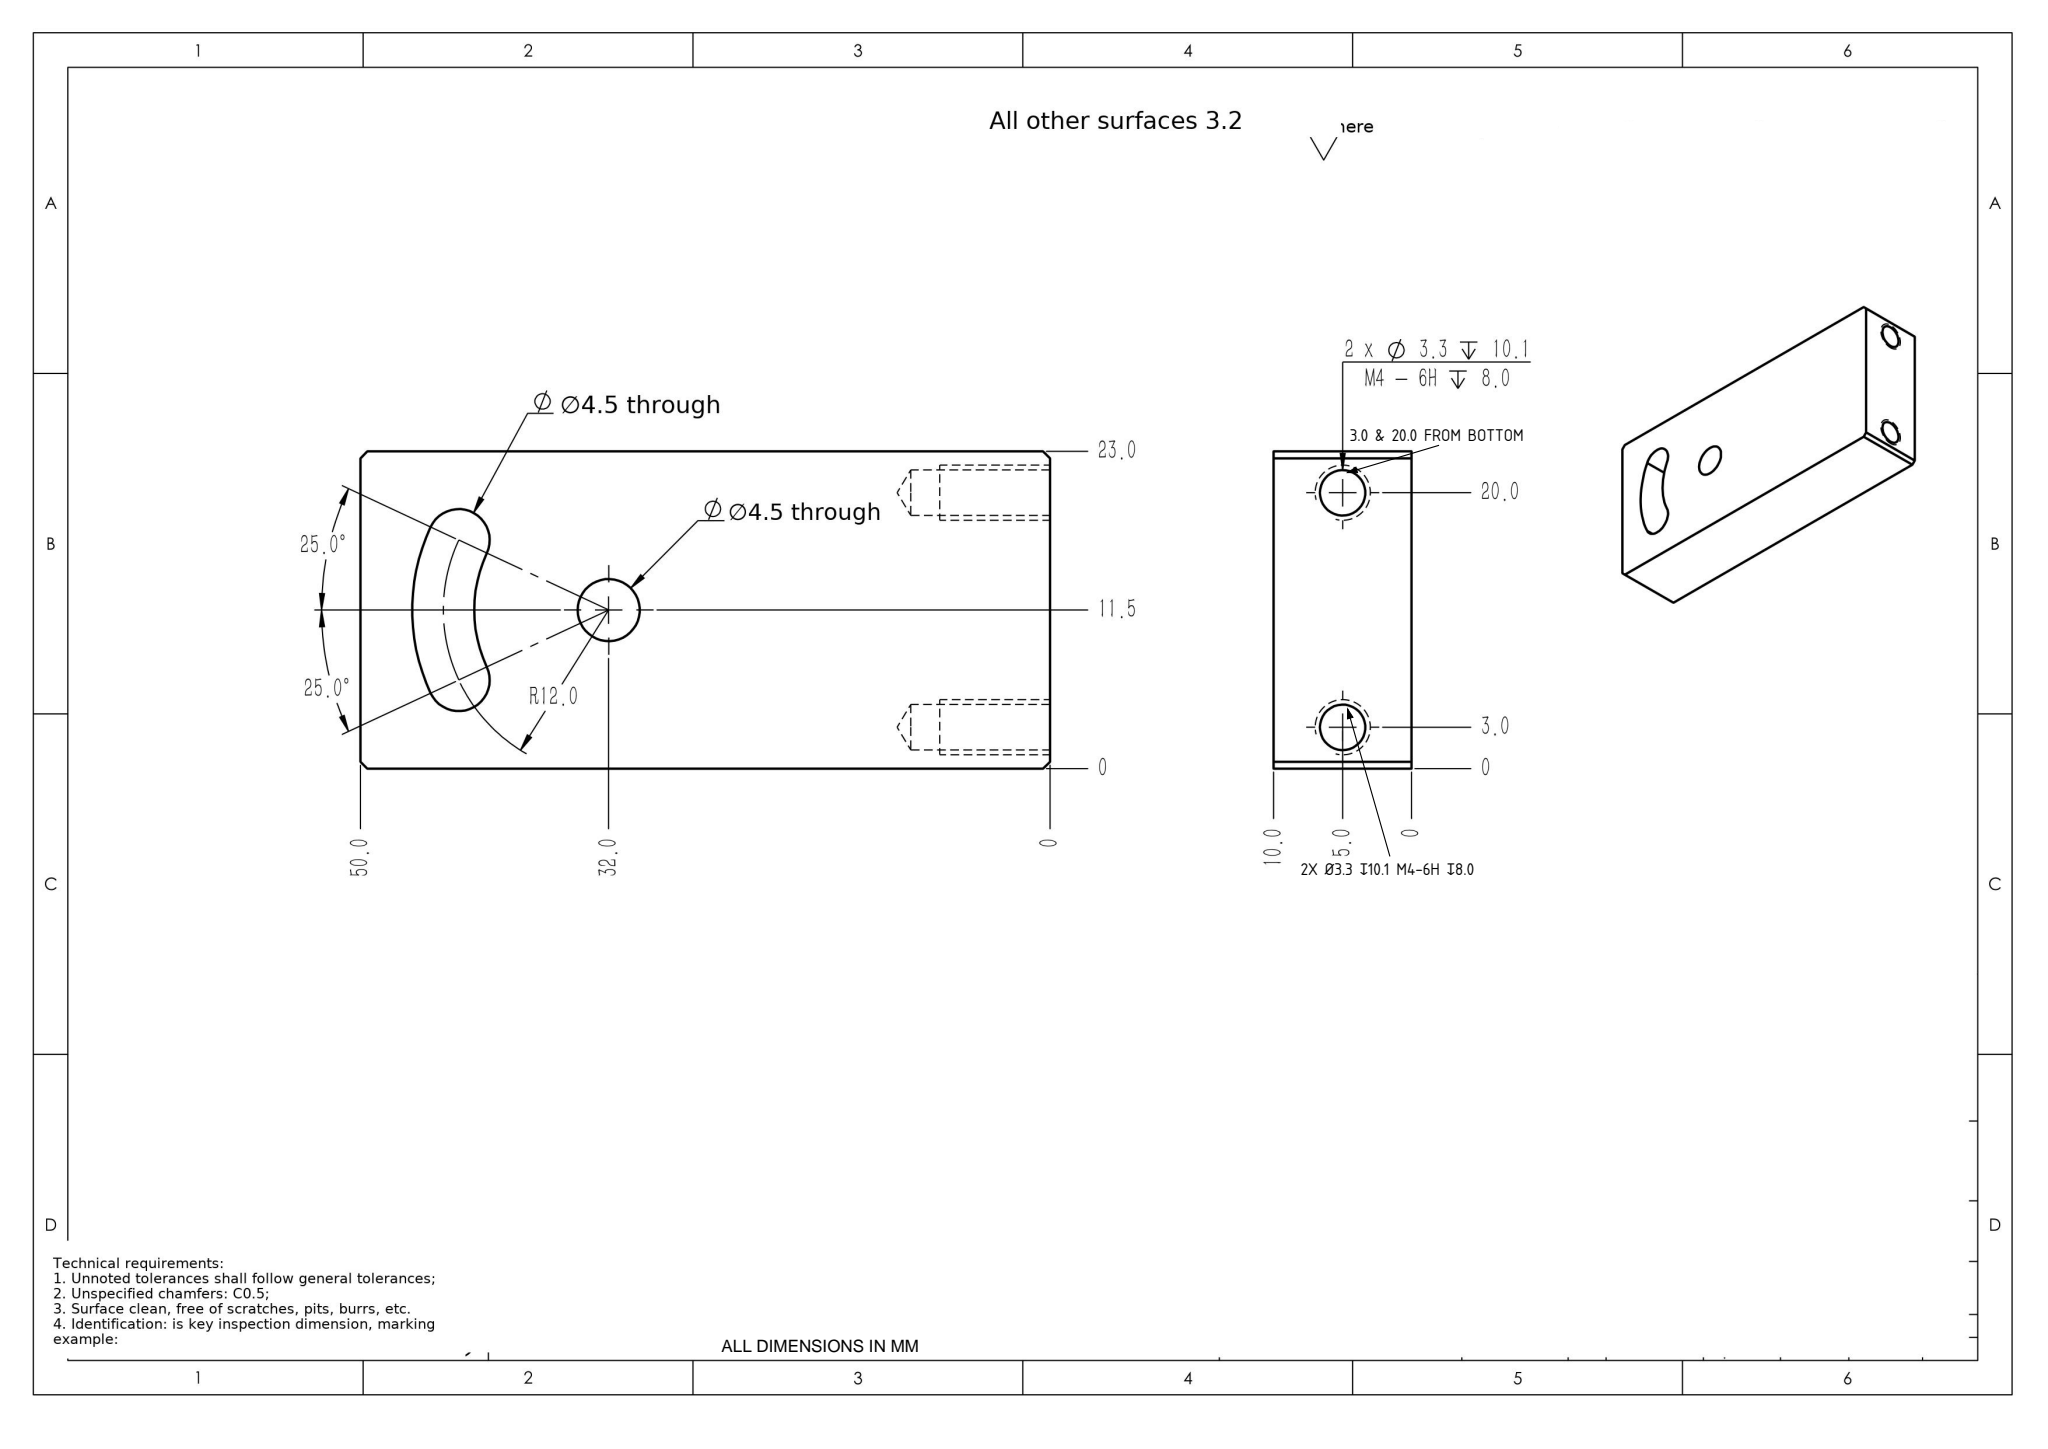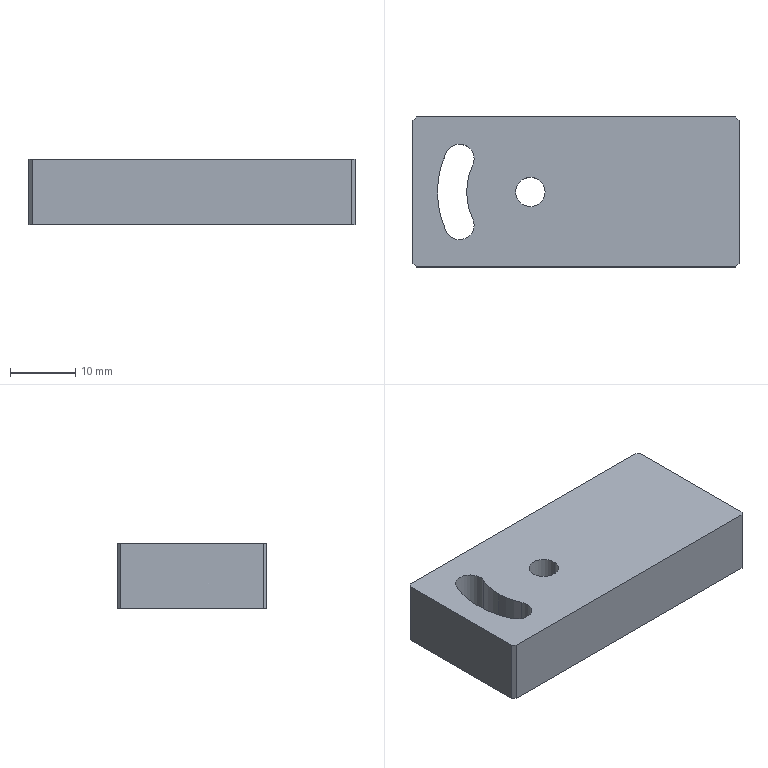Part | SolidWorks | mm | material POM | 1 solid | 26 faces | box 50 x 23 x 10 mm | volume 10527 mm3 | cylinder 12 | plane 10 | cone 4 | commonest cylinder face diameters 4.5 x4 3.3 x4 19.5 x2 28.5 x2
Drawing notes:
2X Ø3.3 DP 10.1, M4-6H DP 8.0 IN END FACE (NOT 4X) | from the solid: Only two Ø3.3 x-axis bores exist: at Y20.0/Z5.0 and Y3.0/Z5.0, from X39.9 to X50.0 (depth 10.1); 118° drill points at X38.9
TAPPED HOLES AT 3.0 & 20.0 FROM BOTTOM, 5.0 FROM FACE | from the solid: hole/bore 3.3 axis x at [y=20.0,z=5.0] and [y=3.0,z=5.0]; bbox 50x23x10
build123d program:
from build123d import *

# Parameters (mm, degrees)
SKETCH1_W             = 50
SKETCH1_H             = 23
BOSS_EXTRUDE1_DEPTH   = 10
M4_TAPPED_HOLE1_D     = 3.3
M4_TAPPED_HOLE1_DEPTH = 10.1
M4_TAPPED_HOLE1_TIP   = 0.9914
SKETCH4_R             = 2.25
CUT_EXTRUDE1_DEPTH    = 30.279
CUT_EXTRUDE2_DEPTH    = 30.279
CHAMFER1_SIZE         = 0.5


with BuildPart() as part:
    # Sketch1 → Boss-Extrude1 (new body)
    with BuildSketch(Plane.XY):
        Rectangle(SKETCH1_W, SKETCH1_H)
    extrude(amount=BOSS_EXTRUDE1_DEPTH)

    # M4 Tapped Hole1
    with Locations(Plane(origin=(25, 0, 0), x_dir=(0, 0, -1), z_dir=(1, 0, 0))):
        with Locations((-5, -8.5), (-5, 8.5)):
            Hole(M4_TAPPED_HOLE1_D / 2, depth=M4_TAPPED_HOLE1_DEPTH)
            with Locations((0, 0, -(M4_TAPPED_HOLE1_DEPTH + M4_TAPPED_HOLE1_TIP / 2))):  # 118° drill point
                Cone(0, M4_TAPPED_HOLE1_D / 2, M4_TAPPED_HOLE1_TIP, mode=Mode.SUBTRACT)

    # Sketch4 → Cut-Extrude1 (cut, through all)
    with BuildSketch(Plane(origin=(0, 0, 0), x_dir=(-1, 0, 0), z_dir=(0, 0, -1))):
        with Locations((7, 0)):
            Circle(SKETCH4_R)
    extrude(amount=-CUT_EXTRUDE1_DEPTH, mode=Mode.SUBTRACT)

    # Sketch5 → Cut-Extrude2 (cut, through all)
    with BuildSketch(Plane(origin=(0, 0, 0), x_dir=(-1, 0, 0), z_dir=(0, 0, -1))):
        with BuildLine():
            ThreePointArc((15.837, -4.121), (16.925, -7.111), (19.915, -6.022))
            ThreePointArc((19.915, -6.022), (21.25, 0), (19.915, 6.022))
            ThreePointArc((19.915, 6.022), (16.925, 7.111), (15.837, 4.121))
            ThreePointArc((15.837, 4.121), (16.75, 0), (15.837, -4.121))
        make_face()
    extrude(amount=-CUT_EXTRUDE2_DEPTH, mode=Mode.SUBTRACT)

    # Chamfer1
    chamfer1_edges = [part.edges().sort_by_distance(p)[0] for p in [
        (25, -11.5, 5),
        (25, 11.5, 5),
        (-25, 11.5, 5),
        (-25, -11.5, 5),
    ]]
    chamfer(chamfer1_edges, length=CHAMFER1_SIZE)


solid = part.part
STEP:
#1=CARTESIAN_POINT('',(-16.75,0.,10.));
#2=VERTEX_POINT('',#1);
#3=CARTESIAN_POINT('',(-15.837,-4.121,10.));
#4=VERTEX_POINT('',#3);
#5=CARTESIAN_POINT('',(-7.,0.,10.));
#6=DIRECTION('',(0.,0.,1.));
#7=DIRECTION('',(-1.,0.,0.));
#8=AXIS2_PLACEMENT_3D('',#5,#6,#7);
#9=CIRCLE('',#8,9.75);
#10=EDGE_CURVE('',#2,#4,#9,.T.);
#11=ORIENTED_EDGE('',*,*,#10,.F.);
#12=CARTESIAN_POINT('',(-16.75,0.,0.));
#13=VERTEX_POINT('',#12);
#14=CARTESIAN_POINT('',(-16.75,0.,10.));
#15=DIRECTION('',(0.,0.,-1.));
#16=VECTOR('',#15,1000.);
#17=LINE('',#14,#16);
#18=EDGE_CURVE('',#2,#13,#17,.T.);
#19=ORIENTED_EDGE('',*,*,#18,.T.);
#20=CARTESIAN_POINT('',(-15.837,-4.121,0.));
#21=VERTEX_POINT('',#20);
#22=CARTESIAN_POINT('',(-7.,0.,0.));
#23=DIRECTION('',(0.,0.,1.));
#24=DIRECTION('',(-1.,0.,0.));
#25=AXIS2_PLACEMENT_3D('',#22,#23,#24);
#26=CIRCLE('',#25,9.75);
#27=EDGE_CURVE('',#13,#21,#26,.T.);
#28=ORIENTED_EDGE('',*,*,#27,.T.);
#29=CARTESIAN_POINT('',(-15.837,-4.121,10.));
#30=DIRECTION('',(0.,0.,-1.));
#31=VECTOR('',#30,1000.);
#32=LINE('',#29,#31);
#33=EDGE_CURVE('',#4,#21,#32,.T.);
#34=ORIENTED_EDGE('',*,*,#33,.F.);
#35=EDGE_LOOP('',(#11,#19,#28,#34));
#36=FACE_OUTER_BOUND('',#35,.T.);
#37=CARTESIAN_POINT('',(-7.,0.,10.));
#38=DIRECTION('',(0.,0.,-1.));
#39=DIRECTION('',(-1.,0.,0.));
#40=AXIS2_PLACEMENT_3D('',#37,#38,#39);
#41=CYLINDRICAL_SURFACE('',#40,9.75);
#42=ADVANCED_FACE('',(#36),#41,.T.);
#43=CARTESIAN_POINT('',(-21.25,0.,10.));
#44=VERTEX_POINT('',#43);
#45=CARTESIAN_POINT('',(-19.915,6.022,10.));
#46=VERTEX_POINT('',#45);
#47=CARTESIAN_POINT('',(-7.,0.,10.));
#48=DIRECTION('',(0.,0.,-1.));
#49=DIRECTION('',(-1.,0.,0.));
#50=AXIS2_PLACEMENT_3D('',#47,#48,#49);
#51=CIRCLE('',#50,14.25);
#52=EDGE_CURVE('',#44,#46,#51,.T.);
#53=ORIENTED_EDGE('',*,*,#52,.F.);
#54=CARTESIAN_POINT('',(-21.25,0.,0.));
#55=VERTEX_POINT('',#54);
#56=CARTESIAN_POINT('',(-21.25,0.,10.));
#57=DIRECTION('',(0.,0.,-1.));
#58=VECTOR('',#57,1000.);
#59=LINE('',#56,#58);
#60=EDGE_CURVE('',#44,#55,#59,.T.);
#61=ORIENTED_EDGE('',*,*,#60,.T.);
#62=CARTESIAN_POINT('',(-19.915,6.022,0.));
#63=VERTEX_POINT('',#62);
#64=CARTESIAN_POINT('',(-7.,0.,0.));
#65=DIRECTION('',(0.,0.,-1.));
#66=DIRECTION('',(-1.,0.,0.));
#67=AXIS2_PLACEMENT_3D('',#64,#65,#66);
#68=CIRCLE('',#67,14.25);
#69=EDGE_CURVE('',#55,#63,#68,.T.);
#70=ORIENTED_EDGE('',*,*,#69,.T.);
#71=CARTESIAN_POINT('',(-19.915,6.022,10.));
#72=DIRECTION('',(0.,0.,-1.));
#73=VECTOR('',#72,1000.);
#74=LINE('',#71,#73);
#75=EDGE_CURVE('',#46,#63,#74,.T.);
#76=ORIENTED_EDGE('',*,*,#75,.F.);
#77=EDGE_LOOP('',(#53,#61,#70,#76));
#78=FACE_OUTER_BOUND('',#77,.T.);
#79=CARTESIAN_POINT('',(-7.,0.,10.));
#80=DIRECTION('',(0.,0.,-1.));
#81=DIRECTION('',(-1.,0.,0.));
#82=AXIS2_PLACEMENT_3D('',#79,#80,#81);
#83=CYLINDRICAL_SURFACE('',#82,14.25);
#84=ADVANCED_FACE('',(#78),#83,.F.);
#85=CARTESIAN_POINT('',(-4.75,0.,10.));
#86=VERTEX_POINT('',#85);
#87=CARTESIAN_POINT('',(-9.25,0.,10.));
#88=VERTEX_POINT('',#87);
#89=CARTESIAN_POINT('',(-7.,0.,10.));
#90=DIRECTION('',(0.,0.,-1.));
#91=DIRECTION('',(-1.,0.,0.));
#92=AXIS2_PLACEMENT_3D('',#89,#90,#91);
#93=CIRCLE('',#92,2.25);
#94=EDGE_CURVE('',#86,#88,#93,.T.);
#95=ORIENTED_EDGE('',*,*,#94,.F.);
#96=CARTESIAN_POINT('',(-4.75,0.,0.));
#97=VERTEX_POINT('',#96);
#98=CARTESIAN_POINT('',(-4.75,0.,10.));
#99=DIRECTION('',(0.,0.,-1.));
#100=VECTOR('',#99,1000.);
#101=LINE('',#98,#100);
#102=EDGE_CURVE('',#86,#97,#101,.T.);
#103=ORIENTED_EDGE('',*,*,#102,.T.);
#104=CARTESIAN_POINT('',(-9.25,0.,0.));
#105=VERTEX_POINT('',#104);
#106=CARTESIAN_POINT('',(-7.,0.,0.));
#107=DIRECTION('',(0.,0.,-1.));
#108=DIRECTION('',(-1.,0.,0.));
#109=AXIS2_PLACEMENT_3D('',#106,#107,#108);
#110=CIRCLE('',#109,2.25);
#111=EDGE_CURVE('',#97,#105,#110,.T.);
#112=ORIENTED_EDGE('',*,*,#111,.T.);
#113=CARTESIAN_POINT('',(-9.25,0.,10.));
#114=DIRECTION('',(0.,0.,-1.));
#115=VECTOR('',#114,1000.);
#116=LINE('',#113,#115);
#117=EDGE_CURVE('',#88,#105,#116,.T.);
#118=ORIENTED_EDGE('',*,*,#117,.F.);
#119=EDGE_LOOP('',(#95,#103,#112,#118));
#120=FACE_OUTER_BOUND('',#119,.T.);
#121=CARTESIAN_POINT('',(-7.,0.,10.));
#122=DIRECTION('',(0.,0.,-1.));
#123=DIRECTION('',(-1.,0.,0.));
#124=AXIS2_PLACEMENT_3D('',#121,#122,#123);
#125=CYLINDRICAL_SURFACE('',#124,2.25);
#126=ADVANCED_FACE('',(#120),#125,.F.);
#127=CARTESIAN_POINT('',(14.9,-8.5,6.65));
#128=VERTEX_POINT('',#127);
#129=CARTESIAN_POINT('',(14.9,-8.5,3.35));
#130=VERTEX_POINT('',#129);
#131=CARTESIAN_POINT('',(14.9,-8.5,5.));
#132=DIRECTION('',(1.,0.,0.));
#133=DIRECTION('',(0.,0.,-1.));
#134=AXIS2_PLACEMENT_3D('',#131,#132,#133);
#135=CIRCLE('',#134,1.65);
#136=EDGE_CURVE('',#128,#130,#135,.T.);
#137=ORIENTED_EDGE('',*,*,#136,.F.);
#138=CARTESIAN_POINT('',(25.,-8.5,6.65));
#139=VERTEX_POINT('',#138);
#140=CARTESIAN_POINT('',(25.,-8.5,6.65));
#141=DIRECTION('',(1.,0.,0.));
#142=VECTOR('',#141,1000.);
#143=LINE('',#140,#142);
#144=EDGE_CURVE('',#128,#139,#143,.T.);
#145=ORIENTED_EDGE('',*,*,#144,.T.);
#146=CARTESIAN_POINT('',(25.,-8.5,3.35));
#147=VERTEX_POINT('',#146);
#148=CARTESIAN_POINT('',(25.,-8.5,5.));
#149=DIRECTION('',(1.,0.,0.));
#150=DIRECTION('',(0.,0.,-1.));
#151=AXIS2_PLACEMENT_3D('',#148,#149,#150);
#152=CIRCLE('',#151,1.65);
#153=EDGE_CURVE('',#139,#147,#152,.T.);
#154=ORIENTED_EDGE('',*,*,#153,.T.);
#155=CARTESIAN_POINT('',(25.,-8.5,3.35));
#156=DIRECTION('',(1.,0.,0.));
#157=VECTOR('',#156,1000.);
#158=LINE('',#155,#157);
#159=EDGE_CURVE('',#130,#147,#158,.T.);
#160=ORIENTED_EDGE('',*,*,#159,.F.);
#161=EDGE_LOOP('',(#137,#145,#154,#160));
#162=FACE_OUTER_BOUND('',#161,.T.);
#163=CARTESIAN_POINT('',(25.,-8.5,5.));
#164=DIRECTION('',(1.,0.,0.));
#165=DIRECTION('',(0.,0.,-1.));
#166=AXIS2_PLACEMENT_3D('',#163,#164,#165);
#167=CYLINDRICAL_SURFACE('',#166,1.65);
#168=ADVANCED_FACE('',(#162),#167,.F.);
#169=CARTESIAN_POINT('',(13.909,-8.5,5.));
#170=VERTEX_POINT('',#169);
#171=CARTESIAN_POINT('',(14.9,-8.5,3.35));
#172=DIRECTION('',(0.515,0.,-0.8572));
#173=VECTOR('',#172,1000.);
#174=LINE('',#171,#173);
#175=EDGE_CURVE('',#170,#130,#174,.T.);
#176=ORIENTED_EDGE('',*,*,#175,.F.);
#177=CARTESIAN_POINT('',(14.9,-8.5,6.65));
#178=DIRECTION('',(0.515,0.,0.8572));
#179=VECTOR('',#178,1000.);
#180=LINE('',#177,#179);
#181=EDGE_CURVE('',#170,#128,#180,.T.);
#182=ORIENTED_EDGE('',*,*,#181,.T.);
#183=ORIENTED_EDGE('',*,*,#136,.T.);
#184=EDGE_LOOP('',(#176,#182,#183));
#185=FACE_OUTER_BOUND('',#184,.T.);
#186=CARTESIAN_POINT('',(14.9,-8.5,5.));
#187=DIRECTION('',(1.,0.,0.));
#188=DIRECTION('',(0.,0.,-1.));
#189=AXIS2_PLACEMENT_3D('',#186,#187,#188);
#190=CONICAL_SURFACE('',#189,1.65,1.03);
#191=ADVANCED_FACE('',(#185),#190,.F.);
#192=CARTESIAN_POINT('',(14.9,8.5,6.65));
#193=VERTEX_POINT('',#192);
#194=CARTESIAN_POINT('',(14.9,8.5,3.35));
#195=VERTEX_POINT('',#194);
#196=CARTESIAN_POINT('',(14.9,8.5,5.));
#197=DIRECTION('',(1.,0.,0.));
#198=DIRECTION('',(0.,0.,-1.));
#199=AXIS2_PLACEMENT_3D('',#196,#197,#198);
#200=CIRCLE('',#199,1.65);
#201=EDGE_CURVE('',#193,#195,#200,.T.);
#202=ORIENTED_EDGE('',*,*,#201,.F.);
#203=CARTESIAN_POINT('',(25.,8.5,6.65));
#204=VERTEX_POINT('',#203);
#205=CARTESIAN_POINT('',(25.,8.5,6.65));
#206=DIRECTION('',(1.,0.,0.));
#207=VECTOR('',#206,1000.);
#208=LINE('',#205,#207);
#209=EDGE_CURVE('',#193,#204,#208,.T.);
#210=ORIENTED_EDGE('',*,*,#209,.T.);
#211=CARTESIAN_POINT('',(25.,8.5,3.35));
#212=VERTEX_POINT('',#211);
#213=CARTESIAN_POINT('',(25.,8.5,5.));
#214=DIRECTION('',(1.,0.,0.));
#215=DIRECTION('',(0.,0.,-1.));
#216=AXIS2_PLACEMENT_3D('',#213,#214,#215);
#217=CIRCLE('',#216,1.65);
#218=EDGE_CURVE('',#204,#212,#217,.T.);
#219=ORIENTED_EDGE('',*,*,#218,.T.);
#220=CARTESIAN_POINT('',(25.,8.5,3.35));
#221=DIRECTION('',(1.,0.,0.));
#222=VECTOR('',#221,1000.);
#223=LINE('',#220,#222);
#224=EDGE_CURVE('',#195,#212,#223,.T.);
#225=ORIENTED_EDGE('',*,*,#224,.F.);
#226=EDGE_LOOP('',(#202,#210,#219,#225));
#227=FACE_OUTER_BOUND('',#226,.T.);
#228=CARTESIAN_POINT('',(25.,8.5,5.));
#229=DIRECTION('',(1.,0.,0.));
#230=DIRECTION('',(0.,0.,-1.));
#231=AXIS2_PLACEMENT_3D('',#228,#229,#230);
#232=CYLINDRICAL_SURFACE('',#231,1.65);
#233=ADVANCED_FACE('',(#227),#232,.F.);
#234=CARTESIAN_POINT('',(13.909,8.5,5.));
#235=VERTEX_POINT('',#234);
#236=CARTESIAN_POINT('',(14.9,8.5,3.35));
#237=DIRECTION('',(0.515,0.,-0.8572));
#238=VECTOR('',#237,1000.);
#239=LINE('',#236,#238);
#240=EDGE_CURVE('',#235,#195,#239,.T.);
#241=ORIENTED_EDGE('',*,*,#240,.F.);
#242=CARTESIAN_POINT('',(14.9,8.5,6.65));
#243=DIRECTION('',(0.515,0.,0.8572));
#244=VECTOR('',#243,1000.);
#245=LINE('',#242,#244);
#246=EDGE_CURVE('',#235,#193,#245,.T.);
#247=ORIENTED_EDGE('',*,*,#246,.T.);
#248=ORIENTED_EDGE('',*,*,#201,.T.);
#249=EDGE_LOOP('',(#241,#247,#248));
#250=FACE_OUTER_BOUND('',#249,.T.);
#251=CARTESIAN_POINT('',(14.9,8.5,5.));
#252=DIRECTION('',(1.,0.,0.));
#253=DIRECTION('',(0.,0.,-1.));
#254=AXIS2_PLACEMENT_3D('',#251,#252,#253);
#255=CONICAL_SURFACE('',#254,1.65,1.03);
#256=ADVANCED_FACE('',(#250),#255,.F.);
#257=CARTESIAN_POINT('',(24.5,-11.5,0.));
#258=VERTEX_POINT('',#257);
#259=CARTESIAN_POINT('',(-24.5,-11.5,0.));
#260=VERTEX_POINT('',#259);
#261=CARTESIAN_POINT('',(25.,-11.5,0.));
#262=DIRECTION('',(-1.,-0.,0.));
#263=VECTOR('',#262,1000.);
#264=LINE('',#261,#263);
#265=EDGE_CURVE('',#258,#260,#264,.T.);
#266=ORIENTED_EDGE('',*,*,#265,.F.);
#267=CARTESIAN_POINT('',(24.5,-11.5,10.));
#268=VERTEX_POINT('',#267);
#269=CARTESIAN_POINT('',(24.5,-11.5,10.));
#270=DIRECTION('',(0.,0.,1.));
#271=VECTOR('',#270,1000.);
#272=LINE('',#269,#271);
#273=EDGE_CURVE('',#258,#268,#272,.T.);
#274=ORIENTED_EDGE('',*,*,#273,.T.);
#275=CARTESIAN_POINT('',(-24.5,-11.5,10.));
#276=VERTEX_POINT('',#275);
#277=CARTESIAN_POINT('',(25.,-11.5,10.));
#278=DIRECTION('',(-1.,-0.,0.));
#279=VECTOR('',#278,1000.);
#280=LINE('',#277,#279);
#281=EDGE_CURVE('',#268,#276,#280,.T.);
#282=ORIENTED_EDGE('',*,*,#281,.T.);
#283=CARTESIAN_POINT('',(-24.5,-11.5,10.));
#284=DIRECTION('',(0.,0.,-1.));
#285=VECTOR('',#284,1000.);
#286=LINE('',#283,#285);
#287=EDGE_CURVE('',#276,#260,#286,.T.);
#288=ORIENTED_EDGE('',*,*,#287,.T.);
#289=EDGE_LOOP('',(#266,#274,#282,#288));
#290=FACE_OUTER_BOUND('',#289,.T.);
#291=CARTESIAN_POINT('',(25.,-11.5,10.));
#292=DIRECTION('',(0.,-1.,0.));
#293=DIRECTION('',(1.,0.,0.));
#294=AXIS2_PLACEMENT_3D('',#291,#292,#293);
#295=PLANE('',#294);
#296=ADVANCED_FACE('',(#290),#295,.T.);
#297=CARTESIAN_POINT('',(25.,-8.5,5.));
#298=DIRECTION('',(1.,0.,0.));
#299=DIRECTION('',(0.,0.,-1.));
#300=AXIS2_PLACEMENT_3D('',#297,#298,#299);
#301=CIRCLE('',#300,1.65);
#302=EDGE_CURVE('',#147,#139,#301,.T.);
#303=ORIENTED_EDGE('',*,*,#302,.F.);
#304=ORIENTED_EDGE('',*,*,#153,.F.);
#305=EDGE_LOOP('',(#303,#304));
#306=FACE_BOUND('',#305,.T.);
#307=CARTESIAN_POINT('',(25.,8.5,5.));
#308=DIRECTION('',(1.,0.,0.));
#309=DIRECTION('',(0.,0.,-1.));
#310=AXIS2_PLACEMENT_3D('',#307,#308,#309);
#311=CIRCLE('',#310,1.65);
#312=EDGE_CURVE('',#212,#204,#311,.T.);
#313=ORIENTED_EDGE('',*,*,#312,.F.);
#314=ORIENTED_EDGE('',*,*,#218,.F.);
#315=EDGE_LOOP('',(#313,#314));
#316=FACE_BOUND('',#315,.T.);
#317=CARTESIAN_POINT('',(25.,-11.,0.));
#318=VERTEX_POINT('',#317);
#319=CARTESIAN_POINT('',(25.,11.,0.));
#320=VERTEX_POINT('',#319);
#321=CARTESIAN_POINT('',(25.,-11.5,0.));
#322=DIRECTION('',(0.,1.,0.));
#323=VECTOR('',#322,1000.);
#324=LINE('',#321,#323);
#325=EDGE_CURVE('',#318,#320,#324,.T.);
#326=ORIENTED_EDGE('',*,*,#325,.T.);
#327=CARTESIAN_POINT('',(25.,11.,10.));
#328=VERTEX_POINT('',#327);
#329=CARTESIAN_POINT('',(25.,11.,10.));
#330=DIRECTION('',(0.,0.,1.));
#331=VECTOR('',#330,1000.);
#332=LINE('',#329,#331);
#333=EDGE_CURVE('',#320,#328,#332,.T.);
#334=ORIENTED_EDGE('',*,*,#333,.T.);
#335=CARTESIAN_POINT('',(25.,-11.,10.));
#336=VERTEX_POINT('',#335);
#337=CARTESIAN_POINT('',(25.,-11.5,10.));
#338=DIRECTION('',(0.,1.,0.));
#339=VECTOR('',#338,1000.);
#340=LINE('',#337,#339);
#341=EDGE_CURVE('',#336,#328,#340,.T.);
#342=ORIENTED_EDGE('',*,*,#341,.F.);
#343=CARTESIAN_POINT('',(25.,-11.,0.));
#344=DIRECTION('',(0.,0.,-1.));
#345=VECTOR('',#344,1000.);
#346=LINE('',#343,#345);
#347=EDGE_CURVE('',#336,#318,#346,.T.);
#348=ORIENTED_EDGE('',*,*,#347,.T.);
#349=EDGE_LOOP('',(#326,#334,#342,#348));
#350=FACE_OUTER_BOUND('',#349,.T.);
#351=CARTESIAN_POINT('',(25.,-11.5,10.));
#352=DIRECTION('',(-1.,0.,0.));
#353=DIRECTION('',(0.,0.,1.));
#354=AXIS2_PLACEMENT_3D('',#351,#352,#353);
#355=PLANE('',#354);
#356=ADVANCED_FACE('',(#306,#316,#350),#355,.F.);
#357=CARTESIAN_POINT('',(24.5,11.5,10.));
#358=VERTEX_POINT('',#357);
#359=CARTESIAN_POINT('',(-24.5,11.5,10.));
#360=VERTEX_POINT('',#359);
#361=CARTESIAN_POINT('',(25.,11.5,10.));
#362=DIRECTION('',(-1.,-0.,0.));
#363=VECTOR('',#362,1000.);
#364=LINE('',#361,#363);
#365=EDGE_CURVE('',#358,#360,#364,.T.);
#366=ORIENTED_EDGE('',*,*,#365,.F.);
#367=CARTESIAN_POINT('',(24.5,11.5,0.));
#368=VERTEX_POINT('',#367);
#369=CARTESIAN_POINT('',(24.5,11.5,10.));
#370=DIRECTION('',(0.,0.,-1.));
#371=VECTOR('',#370,1000.);
#372=LINE('',#369,#371);
#373=EDGE_CURVE('',#358,#368,#372,.T.);
#374=ORIENTED_EDGE('',*,*,#373,.T.);
#375=CARTESIAN_POINT('',(-24.5,11.5,0.));
#376=VERTEX_POINT('',#375);
#377=CARTESIAN_POINT('',(25.,11.5,0.));
#378=DIRECTION('',(-1.,-0.,0.));
#379=VECTOR('',#378,1000.);
#380=LINE('',#377,#379);
#381=EDGE_CURVE('',#368,#376,#380,.T.);
#382=ORIENTED_EDGE('',*,*,#381,.T.);
#383=CARTESIAN_POINT('',(-24.5,11.5,10.));
#384=DIRECTION('',(0.,0.,1.));
#385=VECTOR('',#384,1000.);
#386=LINE('',#383,#385);
#387=EDGE_CURVE('',#376,#360,#386,.T.);
#388=ORIENTED_EDGE('',*,*,#387,.T.);
#389=EDGE_LOOP('',(#366,#374,#382,#388));
#390=FACE_OUTER_BOUND('',#389,.T.);
#391=CARTESIAN_POINT('',(25.,11.5,10.));
#392=DIRECTION('',(0.,-1.,0.));
#393=DIRECTION('',(1.,0.,0.));
#394=AXIS2_PLACEMENT_3D('',#391,#392,#393);
#395=PLANE('',#394);
#396=ADVANCED_FACE('',(#390),#395,.F.);
#397=CARTESIAN_POINT('',(-25.,-11.,10.));
#398=VERTEX_POINT('',#397);
#399=CARTESIAN_POINT('',(-25.,11.,10.));
#400=VERTEX_POINT('',#399);
#401=CARTESIAN_POINT('',(-25.,-11.5,10.));
#402=DIRECTION('',(0.,1.,0.));
#403=VECTOR('',#402,1000.);
#404=LINE('',#401,#403);
#405=EDGE_CURVE('',#398,#400,#404,.T.);
#406=ORIENTED_EDGE('',*,*,#405,.T.);
#407=CARTESIAN_POINT('',(-25.,11.,0.));
#408=VERTEX_POINT('',#407);
#409=CARTESIAN_POINT('',(-25.,11.,0.));
#410=DIRECTION('',(0.,0.,-1.));
#411=VECTOR('',#410,1000.);
#412=LINE('',#409,#411);
#413=EDGE_CURVE('',#400,#408,#412,.T.);
#414=ORIENTED_EDGE('',*,*,#413,.T.);
#415=CARTESIAN_POINT('',(-25.,-11.,0.));
#416=VERTEX_POINT('',#415);
#417=CARTESIAN_POINT('',(-25.,-11.5,0.));
#418=DIRECTION('',(0.,1.,0.));
#419=VECTOR('',#418,1000.);
#420=LINE('',#417,#419);
#421=EDGE_CURVE('',#416,#408,#420,.T.);
#422=ORIENTED_EDGE('',*,*,#421,.F.);
#423=CARTESIAN_POINT('',(-25.,-11.,10.));
#424=DIRECTION('',(0.,0.,1.));
#425=VECTOR('',#424,1000.);
#426=LINE('',#423,#425);
#427=EDGE_CURVE('',#416,#398,#426,.T.);
#428=ORIENTED_EDGE('',*,*,#427,.T.);
#429=EDGE_LOOP('',(#406,#414,#422,#428));
#430=FACE_OUTER_BOUND('',#429,.T.);
#431=CARTESIAN_POINT('',(-25.,-11.5,10.));
#432=DIRECTION('',(-1.,0.,0.));
#433=DIRECTION('',(0.,0.,1.));
#434=AXIS2_PLACEMENT_3D('',#431,#432,#433);
#435=PLANE('',#434);
#436=ADVANCED_FACE('',(#430),#435,.T.);
#437=CARTESIAN_POINT('',(-19.915,-6.022,10.));
#438=VERTEX_POINT('',#437);
#439=CARTESIAN_POINT('',(-17.876,-5.071,10.));
#440=DIRECTION('',(0.,0.,-1.));
#441=DIRECTION('',(-1.,0.,0.));
#442=AXIS2_PLACEMENT_3D('',#439,#440,#441);
#443=CIRCLE('',#442,2.25);
#444=EDGE_CURVE('',#4,#438,#443,.T.);
#445=ORIENTED_EDGE('',*,*,#444,.T.);
#446=CARTESIAN_POINT('',(-7.,0.,10.));
#447=DIRECTION('',(0.,0.,-1.));
#448=DIRECTION('',(-1.,0.,0.));
#449=AXIS2_PLACEMENT_3D('',#446,#447,#448);
#450=CIRCLE('',#449,14.25);
#451=EDGE_CURVE('',#438,#44,#450,.T.);
#452=ORIENTED_EDGE('',*,*,#451,.T.);
#453=ORIENTED_EDGE('',*,*,#52,.T.);
#454=CARTESIAN_POINT('',(-15.837,4.121,10.));
#455=VERTEX_POINT('',#454);
#456=CARTESIAN_POINT('',(-17.876,5.071,10.));
#457=DIRECTION('',(0.,0.,-1.));
#458=DIRECTION('',(-1.,0.,0.));
#459=AXIS2_PLACEMENT_3D('',#456,#457,#458);
#460=CIRCLE('',#459,2.25);
#461=EDGE_CURVE('',#46,#455,#460,.T.);
#462=ORIENTED_EDGE('',*,*,#461,.T.);
#463=CARTESIAN_POINT('',(-7.,0.,10.));
#464=DIRECTION('',(0.,0.,1.));
#465=DIRECTION('',(-1.,0.,0.));
#466=AXIS2_PLACEMENT_3D('',#463,#464,#465);
#467=CIRCLE('',#466,9.75);
#468=EDGE_CURVE('',#455,#2,#467,.T.);
#469=ORIENTED_EDGE('',*,*,#468,.T.);
#470=ORIENTED_EDGE('',*,*,#10,.T.);
#471=EDGE_LOOP('',(#445,#452,#453,#462,#469,#470));
#472=FACE_BOUND('',#471,.T.);
#473=CARTESIAN_POINT('',(-7.,0.,10.));
#474=DIRECTION('',(0.,0.,-1.));
#475=DIRECTION('',(-1.,0.,0.));
#476=AXIS2_PLACEMENT_3D('',#473,#474,#475);
#477=CIRCLE('',#476,2.25);
#478=EDGE_CURVE('',#88,#86,#477,.T.);
#479=ORIENTED_EDGE('',*,*,#478,.T.);
#480=ORIENTED_EDGE('',*,*,#94,.T.);
#481=EDGE_LOOP('',(#479,#480));
#482=FACE_BOUND('',#481,.T.);
#483=ORIENTED_EDGE('',*,*,#341,.T.);
#484=CARTESIAN_POINT('',(24.5,11.5,10.));
#485=DIRECTION('',(-0.7071,0.7071,0.));
#486=VECTOR('',#485,1000.);
#487=LINE('',#484,#486);
#488=EDGE_CURVE('',#328,#358,#487,.T.);
#489=ORIENTED_EDGE('',*,*,#488,.T.);
#490=ORIENTED_EDGE('',*,*,#365,.T.);
#491=CARTESIAN_POINT('',(-25.,11.,10.));
#492=DIRECTION('',(-0.7071,-0.7071,0.));
#493=VECTOR('',#492,1000.);
#494=LINE('',#491,#493);
#495=EDGE_CURVE('',#360,#400,#494,.T.);
#496=ORIENTED_EDGE('',*,*,#495,.T.);
#497=ORIENTED_EDGE('',*,*,#405,.F.);
#498=CARTESIAN_POINT('',(-24.5,-11.5,10.));
#499=DIRECTION('',(0.7071,-0.7071,0.));
#500=VECTOR('',#499,1000.);
#501=LINE('',#498,#500);
#502=EDGE_CURVE('',#398,#276,#501,.T.);
#503=ORIENTED_EDGE('',*,*,#502,.T.);
#504=ORIENTED_EDGE('',*,*,#281,.F.);
#505=CARTESIAN_POINT('',(25.,-11.,10.));
#506=DIRECTION('',(0.7071,0.7071,0.));
#507=VECTOR('',#506,1000.);
#508=LINE('',#505,#507);
#509=EDGE_CURVE('',#268,#336,#508,.T.);
#510=ORIENTED_EDGE('',*,*,#509,.T.);
#511=EDGE_LOOP('',(#483,#489,#490,#496,#497,#503,#504,#510));
#512=FACE_OUTER_BOUND('',#511,.T.);
#513=CARTESIAN_POINT('',(0.,0.,10.));
#514=DIRECTION('',(0.,0.,-1.));
#515=DIRECTION('',(-1.,0.,0.));
#516=AXIS2_PLACEMENT_3D('',#513,#514,#515);
#517=PLANE('',#516);
#518=ADVANCED_FACE('',(#472,#482,#512),#517,.F.);
#519=CARTESIAN_POINT('',(-19.915,-6.022,0.));
#520=VERTEX_POINT('',#519);
#521=CARTESIAN_POINT('',(-7.,0.,0.));
#522=DIRECTION('',(0.,0.,-1.));
#523=DIRECTION('',(-1.,0.,0.));
#524=AXIS2_PLACEMENT_3D('',#521,#522,#523);
#525=CIRCLE('',#524,14.25);
#526=EDGE_CURVE('',#520,#55,#525,.T.);
#527=ORIENTED_EDGE('',*,*,#526,.F.);
#528=CARTESIAN_POINT('',(-17.876,-5.071,0.));
#529=DIRECTION('',(0.,0.,-1.));
#530=DIRECTION('',(-1.,0.,0.));
#531=AXIS2_PLACEMENT_3D('',#528,#529,#530);
#532=CIRCLE('',#531,2.25);
#533=EDGE_CURVE('',#21,#520,#532,.T.);
#534=ORIENTED_EDGE('',*,*,#533,.F.);
#535=ORIENTED_EDGE('',*,*,#27,.F.);
#536=CARTESIAN_POINT('',(-15.837,4.121,0.));
#537=VERTEX_POINT('',#536);
#538=CARTESIAN_POINT('',(-7.,0.,0.));
#539=DIRECTION('',(0.,0.,1.));
#540=DIRECTION('',(-1.,0.,0.));
#541=AXIS2_PLACEMENT_3D('',#538,#539,#540);
#542=CIRCLE('',#541,9.75);
#543=EDGE_CURVE('',#537,#13,#542,.T.);
#544=ORIENTED_EDGE('',*,*,#543,.F.);
#545=CARTESIAN_POINT('',(-17.876,5.071,0.));
#546=DIRECTION('',(0.,0.,-1.));
#547=DIRECTION('',(-1.,0.,0.));
#548=AXIS2_PLACEMENT_3D('',#545,#546,#547);
#549=CIRCLE('',#548,2.25);
#550=EDGE_CURVE('',#63,#537,#549,.T.);
#551=ORIENTED_EDGE('',*,*,#550,.F.);
#552=ORIENTED_EDGE('',*,*,#69,.F.);
#553=EDGE_LOOP('',(#527,#534,#535,#544,#551,#552));
#554=FACE_BOUND('',#553,.T.);
#555=CARTESIAN_POINT('',(-7.,0.,0.));
#556=DIRECTION('',(0.,0.,-1.));
#557=DIRECTION('',(-1.,0.,0.));
#558=AXIS2_PLACEMENT_3D('',#555,#556,#557);
#559=CIRCLE('',#558,2.25);
#560=EDGE_CURVE('',#105,#97,#559,.T.);
#561=ORIENTED_EDGE('',*,*,#560,.F.);
#562=ORIENTED_EDGE('',*,*,#111,.F.);
#563=EDGE_LOOP('',(#561,#562));
#564=FACE_BOUND('',#563,.T.);
#565=ORIENTED_EDGE('',*,*,#381,.F.);
#566=CARTESIAN_POINT('',(18.,18.,0.));
#567=DIRECTION('',(0.7071,-0.7071,0.));
#568=VECTOR('',#567,1000.);
#569=LINE('',#566,#568);
#570=EDGE_CURVE('',#368,#320,#569,.T.);
#571=ORIENTED_EDGE('',*,*,#570,.T.);
#572=ORIENTED_EDGE('',*,*,#325,.F.);
#573=CARTESIAN_POINT('',(18.,-18.,0.));
#574=DIRECTION('',(-0.7071,-0.7071,0.));
#575=VECTOR('',#574,1000.);
#576=LINE('',#573,#575);
#577=EDGE_CURVE('',#318,#258,#576,.T.);
#578=ORIENTED_EDGE('',*,*,#577,.T.);
#579=ORIENTED_EDGE('',*,*,#265,.T.);
#580=CARTESIAN_POINT('',(-18.,-18.,0.));
#581=DIRECTION('',(-0.7071,0.7071,0.));
#582=VECTOR('',#581,1000.);
#583=LINE('',#580,#582);
#584=EDGE_CURVE('',#260,#416,#583,.T.);
#585=ORIENTED_EDGE('',*,*,#584,.T.);
#586=ORIENTED_EDGE('',*,*,#421,.T.);
#587=CARTESIAN_POINT('',(-18.,18.,0.));
#588=DIRECTION('',(0.7071,0.7071,0.));
#589=VECTOR('',#588,1000.);
#590=LINE('',#587,#589);
#591=EDGE_CURVE('',#408,#376,#590,.T.);
#592=ORIENTED_EDGE('',*,*,#591,.T.);
#593=EDGE_LOOP('',(#565,#571,#572,#578,#579,#585,#586,#592));
#594=FACE_OUTER_BOUND('',#593,.T.);
#595=CARTESIAN_POINT('',(0.,0.,0.));
#596=DIRECTION('',(0.,0.,-1.));
#597=DIRECTION('',(-1.,0.,0.));
#598=AXIS2_PLACEMENT_3D('',#595,#596,#597);
#599=PLANE('',#598);
#600=ADVANCED_FACE('',(#554,#564,#594),#599,.T.);
#601=ORIENTED_EDGE('',*,*,#246,.F.);
#602=ORIENTED_EDGE('',*,*,#240,.T.);
#603=CARTESIAN_POINT('',(14.9,8.5,5.));
#604=DIRECTION('',(1.,0.,0.));
#605=DIRECTION('',(0.,0.,-1.));
#606=AXIS2_PLACEMENT_3D('',#603,#604,#605);
#607=CIRCLE('',#606,1.65);
#608=EDGE_CURVE('',#195,#193,#607,.T.);
#609=ORIENTED_EDGE('',*,*,#608,.T.);
#610=EDGE_LOOP('',(#601,#602,#609));
#611=FACE_OUTER_BOUND('',#610,.T.);
#612=CARTESIAN_POINT('',(14.9,8.5,5.));
#613=DIRECTION('',(1.,0.,0.));
#614=DIRECTION('',(0.,0.,-1.));
#615=AXIS2_PLACEMENT_3D('',#612,#613,#614);
#616=CONICAL_SURFACE('',#615,1.65,1.03);
#617=ADVANCED_FACE('',(#611),#616,.F.);
#618=ORIENTED_EDGE('',*,*,#209,.F.);
#619=ORIENTED_EDGE('',*,*,#608,.F.);
#620=ORIENTED_EDGE('',*,*,#224,.T.);
#621=ORIENTED_EDGE('',*,*,#312,.T.);
#622=EDGE_LOOP('',(#618,#619,#620,#621));
#623=FACE_OUTER_BOUND('',#622,.T.);
#624=CARTESIAN_POINT('',(25.,8.5,5.));
#625=DIRECTION('',(1.,0.,0.));
#626=DIRECTION('',(0.,0.,-1.));
#627=AXIS2_PLACEMENT_3D('',#624,#625,#626);
#628=CYLINDRICAL_SURFACE('',#627,1.65);
#629=ADVANCED_FACE('',(#623),#628,.F.);
#630=ORIENTED_EDGE('',*,*,#181,.F.);
#631=ORIENTED_EDGE('',*,*,#175,.T.);
#632=CARTESIAN_POINT('',(14.9,-8.5,5.));
#633=DIRECTION('',(1.,0.,0.));
#634=DIRECTION('',(0.,0.,-1.));
#635=AXIS2_PLACEMENT_3D('',#632,#633,#634);
#636=CIRCLE('',#635,1.65);
#637=EDGE_CURVE('',#130,#128,#636,.T.);
#638=ORIENTED_EDGE('',*,*,#637,.T.);
#639=EDGE_LOOP('',(#630,#631,#638));
#640=FACE_OUTER_BOUND('',#639,.T.);
#641=CARTESIAN_POINT('',(14.9,-8.5,5.));
#642=DIRECTION('',(1.,0.,0.));
#643=DIRECTION('',(0.,0.,-1.));
#644=AXIS2_PLACEMENT_3D('',#641,#642,#643);
#645=CONICAL_SURFACE('',#644,1.65,1.03);
#646=ADVANCED_FACE('',(#640),#645,.F.);
#647=ORIENTED_EDGE('',*,*,#144,.F.);
#648=ORIENTED_EDGE('',*,*,#637,.F.);
#649=ORIENTED_EDGE('',*,*,#159,.T.);
#650=ORIENTED_EDGE('',*,*,#302,.T.);
#651=EDGE_LOOP('',(#647,#648,#649,#650));
#652=FACE_OUTER_BOUND('',#651,.T.);
#653=CARTESIAN_POINT('',(25.,-8.5,5.));
#654=DIRECTION('',(1.,0.,0.));
#655=DIRECTION('',(0.,0.,-1.));
#656=AXIS2_PLACEMENT_3D('',#653,#654,#655);
#657=CYLINDRICAL_SURFACE('',#656,1.65);
#658=ADVANCED_FACE('',(#652),#657,.F.);
#659=ORIENTED_EDGE('',*,*,#102,.F.);
#660=ORIENTED_EDGE('',*,*,#478,.F.);
#661=ORIENTED_EDGE('',*,*,#117,.T.);
#662=ORIENTED_EDGE('',*,*,#560,.T.);
#663=EDGE_LOOP('',(#659,#660,#661,#662));
#664=FACE_OUTER_BOUND('',#663,.T.);
#665=CARTESIAN_POINT('',(-7.,0.,10.));
#666=DIRECTION('',(0.,0.,-1.));
#667=DIRECTION('',(-1.,0.,0.));
#668=AXIS2_PLACEMENT_3D('',#665,#666,#667);
#669=CYLINDRICAL_SURFACE('',#668,2.25);
#670=ADVANCED_FACE('',(#664),#669,.F.);
#671=ORIENTED_EDGE('',*,*,#60,.F.);
#672=ORIENTED_EDGE('',*,*,#451,.F.);
#673=CARTESIAN_POINT('',(-19.915,-6.022,10.));
#674=DIRECTION('',(0.,0.,-1.));
#675=VECTOR('',#674,1000.);
#676=LINE('',#673,#675);
#677=EDGE_CURVE('',#438,#520,#676,.T.);
#678=ORIENTED_EDGE('',*,*,#677,.T.);
#679=ORIENTED_EDGE('',*,*,#526,.T.);
#680=EDGE_LOOP('',(#671,#672,#678,#679));
#681=FACE_OUTER_BOUND('',#680,.T.);
#682=CARTESIAN_POINT('',(-7.,0.,10.));
#683=DIRECTION('',(0.,0.,-1.));
#684=DIRECTION('',(-1.,0.,0.));
#685=AXIS2_PLACEMENT_3D('',#682,#683,#684);
#686=CYLINDRICAL_SURFACE('',#685,14.25);
#687=ADVANCED_FACE('',(#681),#686,.F.);
#688=ORIENTED_EDGE('',*,*,#533,.T.);
#689=ORIENTED_EDGE('',*,*,#677,.F.);
#690=ORIENTED_EDGE('',*,*,#444,.F.);
#691=ORIENTED_EDGE('',*,*,#33,.T.);
#692=EDGE_LOOP('',(#688,#689,#690,#691));
#693=FACE_OUTER_BOUND('',#692,.T.);
#694=CARTESIAN_POINT('',(-17.876,-5.071,10.));
#695=DIRECTION('',(0.,0.,-1.));
#696=DIRECTION('',(-1.,0.,0.));
#697=AXIS2_PLACEMENT_3D('',#694,#695,#696);
#698=CYLINDRICAL_SURFACE('',#697,2.25);
#699=ADVANCED_FACE('',(#693),#698,.F.);
#700=ORIENTED_EDGE('',*,*,#18,.F.);
#701=ORIENTED_EDGE('',*,*,#468,.F.);
#702=CARTESIAN_POINT('',(-15.837,4.121,10.));
#703=DIRECTION('',(0.,0.,-1.));
#704=VECTOR('',#703,1000.);
#705=LINE('',#702,#704);
#706=EDGE_CURVE('',#455,#537,#705,.T.);
#707=ORIENTED_EDGE('',*,*,#706,.T.);
#708=ORIENTED_EDGE('',*,*,#543,.T.);
#709=EDGE_LOOP('',(#700,#701,#707,#708));
#710=FACE_OUTER_BOUND('',#709,.T.);
#711=CARTESIAN_POINT('',(-7.,0.,10.));
#712=DIRECTION('',(0.,0.,-1.));
#713=DIRECTION('',(-1.,0.,0.));
#714=AXIS2_PLACEMENT_3D('',#711,#712,#713);
#715=CYLINDRICAL_SURFACE('',#714,9.75);
#716=ADVANCED_FACE('',(#710),#715,.T.);
#717=ORIENTED_EDGE('',*,*,#550,.T.);
#718=ORIENTED_EDGE('',*,*,#706,.F.);
#719=ORIENTED_EDGE('',*,*,#461,.F.);
#720=ORIENTED_EDGE('',*,*,#75,.T.);
#721=EDGE_LOOP('',(#717,#718,#719,#720));
#722=FACE_OUTER_BOUND('',#721,.T.);
#723=CARTESIAN_POINT('',(-17.876,5.071,10.));
#724=DIRECTION('',(0.,0.,-1.));
#725=DIRECTION('',(-1.,0.,0.));
#726=AXIS2_PLACEMENT_3D('',#723,#724,#725);
#727=CYLINDRICAL_SURFACE('',#726,2.25);
#728=ADVANCED_FACE('',(#722),#727,.F.);
#729=ORIENTED_EDGE('',*,*,#488,.F.);
#730=ORIENTED_EDGE('',*,*,#333,.F.);
#731=ORIENTED_EDGE('',*,*,#570,.F.);
#732=ORIENTED_EDGE('',*,*,#373,.F.);
#733=EDGE_LOOP('',(#729,#730,#731,#732));
#734=FACE_OUTER_BOUND('',#733,.T.);
#735=CARTESIAN_POINT('',(24.5,11.5,10.));
#736=DIRECTION('',(-0.7071,-0.7071,0.));
#737=DIRECTION('',(0.,0.,-1.));
#738=AXIS2_PLACEMENT_3D('',#735,#736,#737);
#739=PLANE('',#738);
#740=ADVANCED_FACE('',(#734),#739,.F.);
#741=ORIENTED_EDGE('',*,*,#509,.F.);
#742=ORIENTED_EDGE('',*,*,#273,.F.);
#743=ORIENTED_EDGE('',*,*,#577,.F.);
#744=ORIENTED_EDGE('',*,*,#347,.F.);
#745=EDGE_LOOP('',(#741,#742,#743,#744));
#746=FACE_OUTER_BOUND('',#745,.T.);
#747=CARTESIAN_POINT('',(25.,-11.,10.));
#748=DIRECTION('',(0.7071,-0.7071,0.));
#749=DIRECTION('',(0.,0.,1.));
#750=AXIS2_PLACEMENT_3D('',#747,#748,#749);
#751=PLANE('',#750);
#752=ADVANCED_FACE('',(#746),#751,.T.);
#753=ORIENTED_EDGE('',*,*,#495,.F.);
#754=ORIENTED_EDGE('',*,*,#387,.F.);
#755=ORIENTED_EDGE('',*,*,#591,.F.);
#756=ORIENTED_EDGE('',*,*,#413,.F.);
#757=EDGE_LOOP('',(#753,#754,#755,#756));
#758=FACE_OUTER_BOUND('',#757,.T.);
#759=CARTESIAN_POINT('',(-25.,11.,10.));
#760=DIRECTION('',(-0.7071,0.7071,0.));
#761=DIRECTION('',(0.,0.,1.));
#762=AXIS2_PLACEMENT_3D('',#759,#760,#761);
#763=PLANE('',#762);
#764=ADVANCED_FACE('',(#758),#763,.T.);
#765=ORIENTED_EDGE('',*,*,#502,.F.);
#766=ORIENTED_EDGE('',*,*,#427,.F.);
#767=ORIENTED_EDGE('',*,*,#584,.F.);
#768=ORIENTED_EDGE('',*,*,#287,.F.);
#769=EDGE_LOOP('',(#765,#766,#767,#768));
#770=FACE_OUTER_BOUND('',#769,.T.);
#771=CARTESIAN_POINT('',(-24.5,-11.5,10.));
#772=DIRECTION('',(0.7071,0.7071,0.));
#773=DIRECTION('',(0.,0.,-1.));
#774=AXIS2_PLACEMENT_3D('',#771,#772,#773);
#775=PLANE('',#774);
#776=ADVANCED_FACE('',(#770),#775,.F.);
#777=CLOSED_SHELL('',(#42,#84,#126,#168,#191,#233,#256,#296,#356,#396,#436,#518,#600,#617,#629,#646,#658,#670,#687,#699,#716,#728,#740,#752,#764,#776));
#778=MANIFOLD_SOLID_BREP('',#777);
#779=CARTESIAN_POINT('',(0.,0.,0.));
#780=DIRECTION('',(0.,0.,1.));
#781=DIRECTION('',(1.,0.,0.));
#782=AXIS2_PLACEMENT_3D('',#779,#780,#781);
#783=(LENGTH_UNIT()NAMED_UNIT(*)SI_UNIT(.MILLI.,.METRE.));
#784=UNCERTAINTY_MEASURE_WITH_UNIT(LENGTH_MEASURE(0.00001),#783,'','');
#785=(NAMED_UNIT(*)PLANE_ANGLE_UNIT()SI_UNIT($,.RADIAN.));
#786=(NAMED_UNIT(*)SI_UNIT($,.STERADIAN.)SOLID_ANGLE_UNIT());
#787=(GEOMETRIC_REPRESENTATION_CONTEXT(3)GLOBAL_UNCERTAINTY_ASSIGNED_CONTEXT((#784))GLOBAL_UNIT_ASSIGNED_CONTEXT((#783,#785,#786))REPRESENTATION_CONTEXT('',''));
#788=ADVANCED_BREP_SHAPE_REPRESENTATION('',(#778,#782),#787);